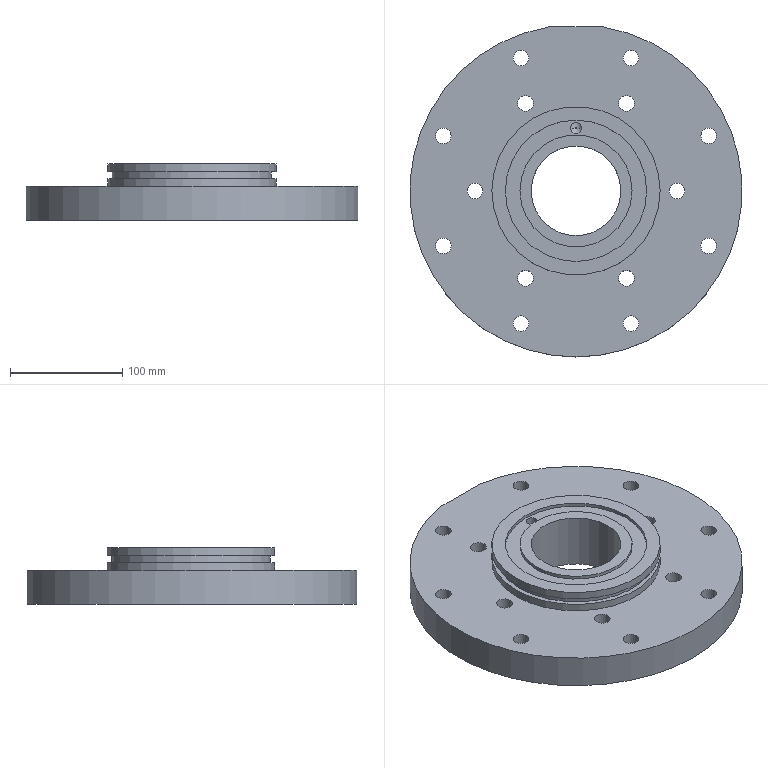Component | NX | CH3404_6-1 | 1 solid | 67 faces | volume 2036318 mm3 | cylinder 38 | plane 22 | cone 7 | commonest cylinder face diameters 14 x14 20 x14 150 x2 10 x2 296 x1 80 x1 100 x1 126 x1